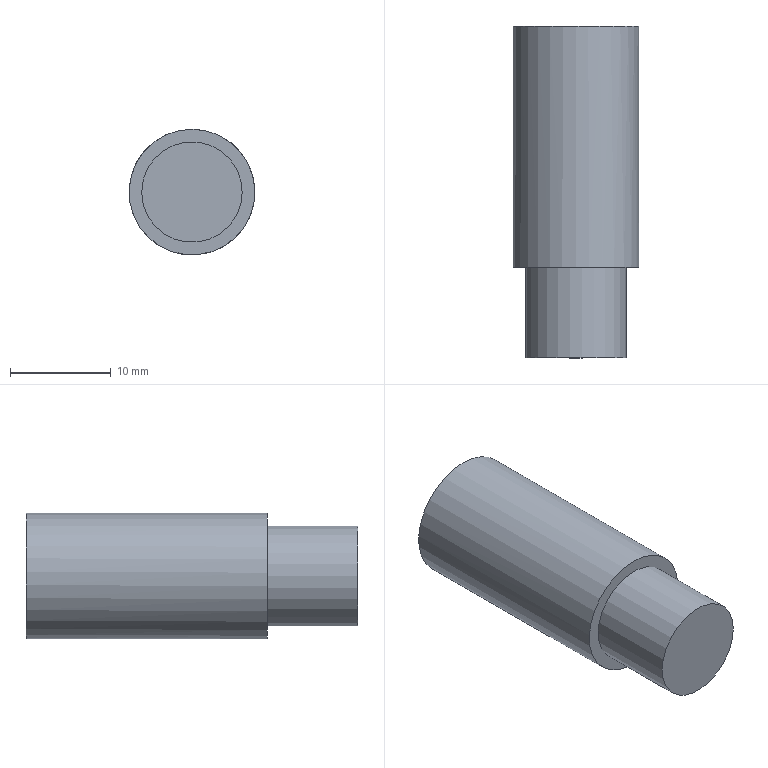Component | NX | SHORT_SHAFT | 1 solid | 5 faces | box 12.5 x 33 x 12.5 mm | volume 3652 mm3 | plane 3 | cylinder 2 | commonest cylinder face diameters 12.5 x1 10 x1
STEP:
#1=CARTESIAN_POINT('',(0.,0.,0.));
#2=DIRECTION('',(0.,0.,1.));
#3=DIRECTION('',(1.,0.,0.));
#4=AXIS2_PLACEMENT_3D('',#1,#2,#3);
#5=CARTESIAN_POINT('',(-126.826,-59.005,96.25));
#6=VERTEX_POINT('',#5);
#7=CARTESIAN_POINT('',(-126.826,-59.005,90.));
#8=DIRECTION('',(0.,1.,0.));
#9=DIRECTION('',(0.,0.,1.));
#10=AXIS2_PLACEMENT_3D('',#7,#8,#9);
#11=CIRCLE('',#10,6.25);
#12=CARTESIAN_POINT('',(-126.826,-68.005,90.));
#13=DIRECTION('',(0.,1.,0.));
#14=DIRECTION('',(0.,0.,1.));
#15=AXIS2_PLACEMENT_3D('',#12,#13,#14);
#16=CYLINDRICAL_SURFACE('',#15,6.25);
#17=CARTESIAN_POINT('',(0.,9.));
#18=DIRECTION('',(1.,0.));
#19=VECTOR('',#18,1.);
#20=LINE('',#17,#19);
#21=(GEOMETRIC_REPRESENTATION_CONTEXT(2)PARAMETRIC_REPRESENTATION_CONTEXT()REPRESENTATION_CONTEXT('',''));
#22=DEFINITIONAL_REPRESENTATION('',(#20),#21);
#23=PCURVE('',#16,#22);
#24=CARTESIAN_POINT('',(-126.826,-59.005,90.));
#25=DIRECTION('',(0.,1.,0.));
#26=DIRECTION('',(0.,0.,1.));
#27=AXIS2_PLACEMENT_3D('',#24,#25,#26);
#28=PLANE('',#27);
#29=CARTESIAN_POINT('',(0.,0.));
#30=DIRECTION('',(1.,0.));
#31=AXIS2_PLACEMENT_2D('',#29,#30);
#32=CIRCLE('',#31,6.25);
#33=(GEOMETRIC_REPRESENTATION_CONTEXT(2)PARAMETRIC_REPRESENTATION_CONTEXT()REPRESENTATION_CONTEXT('',''));
#34=DEFINITIONAL_REPRESENTATION('',(#32),#33);
#35=PCURVE('',#28,#34);
#36=SURFACE_CURVE('',#11,(#23,#35),.PCURVE_S1.);
#37=EDGE_CURVE('',#6,#6,#36,.T.);
#38=ORIENTED_EDGE('',*,*,#37,.T.);
#39=CARTESIAN_POINT('',(-126.826,-35.005,96.25));
#40=VERTEX_POINT('',#39);
#41=CARTESIAN_POINT('',(-126.826,-59.005,96.25));
#42=CARTESIAN_POINT('',(-126.826,-35.005,96.25));
#43=B_SPLINE_CURVE_WITH_KNOTS('',1,(#41,#42),.UNSPECIFIED.,.F.,.F.,(2,2),(9.,33.),.PIECEWISE_BEZIER_KNOTS.);
#44=CARTESIAN_POINT('',(6.283,0.));
#45=DIRECTION('',(0.,1.));
#46=VECTOR('',#45,1.);
#47=LINE('',#44,#46);
#48=(GEOMETRIC_REPRESENTATION_CONTEXT(2)PARAMETRIC_REPRESENTATION_CONTEXT()REPRESENTATION_CONTEXT('',''));
#49=DEFINITIONAL_REPRESENTATION('',(#47),#48);
#50=PCURVE('',#16,#49);
#51=CARTESIAN_POINT('',(0.,0.));
#52=DIRECTION('',(0.,1.));
#53=VECTOR('',#52,1.);
#54=LINE('',#51,#53);
#55=(GEOMETRIC_REPRESENTATION_CONTEXT(2)PARAMETRIC_REPRESENTATION_CONTEXT()REPRESENTATION_CONTEXT('',''));
#56=DEFINITIONAL_REPRESENTATION('',(#54),#55);
#57=PCURVE('',#16,#56);
#58=SEAM_CURVE('',#43,(#50,#57),.PCURVE_S1.);
#59=EDGE_CURVE('',#6,#40,#58,.T.);
#60=ORIENTED_EDGE('',*,*,#59,.T.);
#61=CARTESIAN_POINT('',(-120.576,-35.005,90.));
#62=VERTEX_POINT('',#61);
#63=CARTESIAN_POINT('',(-126.826,-35.005,90.));
#64=DIRECTION('',(0.,-1.,0.));
#65=DIRECTION('',(1.,0.,0.));
#66=AXIS2_PLACEMENT_3D('',#63,#64,#65);
#67=CIRCLE('',#66,6.25);
#68=CARTESIAN_POINT('',(7.854,33.));
#69=DIRECTION('',(-1.,0.));
#70=VECTOR('',#69,1.);
#71=LINE('',#68,#70);
#72=(GEOMETRIC_REPRESENTATION_CONTEXT(2)PARAMETRIC_REPRESENTATION_CONTEXT()REPRESENTATION_CONTEXT('',''));
#73=DEFINITIONAL_REPRESENTATION('',(#71),#72);
#74=PCURVE('',#16,#73);
#75=CARTESIAN_POINT('',(-126.826,-35.005,90.));
#76=DIRECTION('',(0.,-1.,0.));
#77=DIRECTION('',(0.,0.,-1.));
#78=AXIS2_PLACEMENT_3D('',#75,#76,#77);
#79=PLANE('',#78);
#80=CARTESIAN_POINT('',(0.,0.));
#81=DIRECTION('',(0.,1.));
#82=AXIS2_PLACEMENT_2D('',#80,#81);
#83=CIRCLE('',#82,6.25);
#84=(GEOMETRIC_REPRESENTATION_CONTEXT(2)PARAMETRIC_REPRESENTATION_CONTEXT()REPRESENTATION_CONTEXT('',''));
#85=DEFINITIONAL_REPRESENTATION('',(#83),#84);
#86=PCURVE('',#79,#85);
#87=SURFACE_CURVE('',#67,(#74,#86),.PCURVE_S1.);
#88=EDGE_CURVE('',#40,#62,#87,.T.);
#89=ORIENTED_EDGE('',*,*,#88,.T.);
#90=CARTESIAN_POINT('',(-126.826,-35.005,90.));
#91=DIRECTION('',(0.,-1.,0.));
#92=DIRECTION('',(1.,0.,0.));
#93=AXIS2_PLACEMENT_3D('',#90,#91,#92);
#94=CIRCLE('',#93,6.25);
#95=CARTESIAN_POINT('',(1.571,33.));
#96=DIRECTION('',(-1.,0.));
#97=VECTOR('',#96,1.);
#98=LINE('',#95,#97);
#99=(GEOMETRIC_REPRESENTATION_CONTEXT(2)PARAMETRIC_REPRESENTATION_CONTEXT()REPRESENTATION_CONTEXT('',''));
#100=DEFINITIONAL_REPRESENTATION('',(#98),#99);
#101=PCURVE('',#16,#100);
#102=CARTESIAN_POINT('',(0.,0.));
#103=DIRECTION('',(0.,1.));
#104=AXIS2_PLACEMENT_2D('',#102,#103);
#105=CIRCLE('',#104,6.25);
#106=(GEOMETRIC_REPRESENTATION_CONTEXT(2)PARAMETRIC_REPRESENTATION_CONTEXT()REPRESENTATION_CONTEXT('',''));
#107=DEFINITIONAL_REPRESENTATION('',(#105),#106);
#108=PCURVE('',#79,#107);
#109=SURFACE_CURVE('',#94,(#101,#108),.PCURVE_S1.);
#110=EDGE_CURVE('',#62,#40,#109,.T.);
#111=ORIENTED_EDGE('',*,*,#110,.T.);
#112=ORIENTED_EDGE('',*,*,#59,.F.);
#113=EDGE_LOOP('',(#38,#60,#89,#111,#112));
#114=FACE_BOUND('',#113,.T.);
#115=ADVANCED_FACE('',(#114),#16,.T.);
#116=ORIENTED_EDGE('',*,*,#110,.F.);
#117=ORIENTED_EDGE('',*,*,#88,.F.);
#118=EDGE_LOOP('',(#116,#117));
#119=FACE_BOUND('',#118,.T.);
#120=ADVANCED_FACE('',(#119),#79,.F.);
#121=CARTESIAN_POINT('',(-121.826,-59.005,90.));
#122=VERTEX_POINT('',#121);
#123=CARTESIAN_POINT('',(-126.826,-59.005,90.));
#124=DIRECTION('',(0.,-1.,0.));
#125=DIRECTION('',(1.,0.,0.));
#126=AXIS2_PLACEMENT_3D('',#123,#124,#125);
#127=CIRCLE('',#126,5.);
#128=CARTESIAN_POINT('',(0.,5.));
#129=CARTESIAN_POINT('',(8.66,5.));
#130=CARTESIAN_POINT('',(4.33,-2.5));
#131=CARTESIAN_POINT('',(0.,-10.));
#132=CARTESIAN_POINT('',(-4.33,-2.5));
#133=CARTESIAN_POINT('',(-8.66,5.));
#134=CARTESIAN_POINT('',(0.,5.));
#135=(BOUNDED_CURVE()B_SPLINE_CURVE(2,(#128,#129,#130,#131,#132,#133,#134),.UNSPECIFIED.,.T.,.F.)B_SPLINE_CURVE_WITH_KNOTS((1,2,2,2,2,1),(-2.094,0.,2.094,4.189,6.283,8.378),.UNSPECIFIED.)CURVE()GEOMETRIC_REPRESENTATION_ITEM()RATIONAL_B_SPLINE_CURVE((1.,0.5,1.,0.5,1.,0.5,1.))REPRESENTATION_ITEM(''));
#136=(GEOMETRIC_REPRESENTATION_CONTEXT(2)PARAMETRIC_REPRESENTATION_CONTEXT()REPRESENTATION_CONTEXT('',''));
#137=DEFINITIONAL_REPRESENTATION('',(#135),#136);
#138=PCURVE('',#28,#137);
#139=CARTESIAN_POINT('',(-126.826,-68.005,90.));
#140=DIRECTION('',(0.,1.,0.));
#141=DIRECTION('',(1.,0.,0.));
#142=AXIS2_PLACEMENT_3D('',#139,#140,#141);
#143=CYLINDRICAL_SURFACE('',#142,5.);
#144=CARTESIAN_POINT('',(6.283,9.));
#145=DIRECTION('',(-1.,0.));
#146=VECTOR('',#145,1.);
#147=LINE('',#144,#146);
#148=(GEOMETRIC_REPRESENTATION_CONTEXT(2)PARAMETRIC_REPRESENTATION_CONTEXT()REPRESENTATION_CONTEXT('',''));
#149=DEFINITIONAL_REPRESENTATION('',(#147),#148);
#150=PCURVE('',#143,#149);
#151=SURFACE_CURVE('',#127,(#138,#150),.PCURVE_S1.);
#152=EDGE_CURVE('',#122,#122,#151,.T.);
#153=ORIENTED_EDGE('',*,*,#152,.F.);
#154=EDGE_LOOP('',(#153));
#155=FACE_BOUND('',#154,.T.);
#156=ORIENTED_EDGE('',*,*,#37,.F.);
#157=EDGE_LOOP('',(#156));
#158=FACE_BOUND('',#157,.T.);
#159=ADVANCED_FACE('',(#155,#158),#28,.F.);
#160=CARTESIAN_POINT('',(-121.826,-68.005,90.));
#161=VERTEX_POINT('',#160);
#162=CARTESIAN_POINT('',(-126.826,-68.005,90.));
#163=DIRECTION('',(0.,1.,0.));
#164=DIRECTION('',(1.,0.,0.));
#165=AXIS2_PLACEMENT_3D('',#162,#163,#164);
#166=CIRCLE('',#165,5.);
#167=CARTESIAN_POINT('',(-126.826,-68.005,90.));
#168=DIRECTION('',(0.,-1.,0.));
#169=DIRECTION('',(0.,0.,-1.));
#170=AXIS2_PLACEMENT_3D('',#167,#168,#169);
#171=PLANE('',#170);
#172=CARTESIAN_POINT('',(0.,5.));
#173=CARTESIAN_POINT('',(8.66,5.));
#174=CARTESIAN_POINT('',(4.33,-2.5));
#175=CARTESIAN_POINT('',(0.,-10.));
#176=CARTESIAN_POINT('',(-4.33,-2.5));
#177=CARTESIAN_POINT('',(-8.66,5.));
#178=CARTESIAN_POINT('',(0.,5.));
#179=(BOUNDED_CURVE()B_SPLINE_CURVE(2,(#172,#173,#174,#175,#176,#177,#178),.UNSPECIFIED.,.T.,.F.)B_SPLINE_CURVE_WITH_KNOTS((1,2,2,2,2,1),(-2.094,0.,2.094,4.189,6.283,8.378),.UNSPECIFIED.)CURVE()GEOMETRIC_REPRESENTATION_ITEM()RATIONAL_B_SPLINE_CURVE((1.,0.5,1.,0.5,1.,0.5,1.))REPRESENTATION_ITEM(''));
#180=(GEOMETRIC_REPRESENTATION_CONTEXT(2)PARAMETRIC_REPRESENTATION_CONTEXT()REPRESENTATION_CONTEXT('',''));
#181=DEFINITIONAL_REPRESENTATION('',(#179),#180);
#182=PCURVE('',#171,#181);
#183=CARTESIAN_POINT('',(0.,0.));
#184=DIRECTION('',(1.,0.));
#185=VECTOR('',#184,1.);
#186=LINE('',#183,#185);
#187=(GEOMETRIC_REPRESENTATION_CONTEXT(2)PARAMETRIC_REPRESENTATION_CONTEXT()REPRESENTATION_CONTEXT('',''));
#188=DEFINITIONAL_REPRESENTATION('',(#186),#187);
#189=PCURVE('',#143,#188);
#190=SURFACE_CURVE('',#166,(#182,#189),.PCURVE_S1.);
#191=EDGE_CURVE('',#161,#161,#190,.T.);
#192=ORIENTED_EDGE('',*,*,#191,.F.);
#193=EDGE_LOOP('',(#192));
#194=FACE_BOUND('',#193,.T.);
#195=ADVANCED_FACE('',(#194),#171,.T.);
#196=ORIENTED_EDGE('',*,*,#152,.T.);
#197=CARTESIAN_POINT('',(-121.826,-68.005,90.));
#198=CARTESIAN_POINT('',(-121.826,-59.005,90.));
#199=B_SPLINE_CURVE_WITH_KNOTS('',1,(#197,#198),.UNSPECIFIED.,.F.,.F.,(2,2),(0.,9.),.PIECEWISE_BEZIER_KNOTS.);
#200=CARTESIAN_POINT('',(0.,0.));
#201=DIRECTION('',(0.,1.));
#202=VECTOR('',#201,1.);
#203=LINE('',#200,#202);
#204=(GEOMETRIC_REPRESENTATION_CONTEXT(2)PARAMETRIC_REPRESENTATION_CONTEXT()REPRESENTATION_CONTEXT('',''));
#205=DEFINITIONAL_REPRESENTATION('',(#203),#204);
#206=PCURVE('',#143,#205);
#207=CARTESIAN_POINT('',(6.283,0.));
#208=DIRECTION('',(0.,1.));
#209=VECTOR('',#208,1.);
#210=LINE('',#207,#209);
#211=(GEOMETRIC_REPRESENTATION_CONTEXT(2)PARAMETRIC_REPRESENTATION_CONTEXT()REPRESENTATION_CONTEXT('',''));
#212=DEFINITIONAL_REPRESENTATION('',(#210),#211);
#213=PCURVE('',#143,#212);
#214=SEAM_CURVE('',#199,(#206,#213),.PCURVE_S1.);
#215=EDGE_CURVE('',#161,#122,#214,.T.);
#216=ORIENTED_EDGE('',*,*,#215,.F.);
#217=ORIENTED_EDGE('',*,*,#191,.T.);
#218=ORIENTED_EDGE('',*,*,#215,.T.);
#219=EDGE_LOOP('',(#196,#216,#217,#218));
#220=FACE_BOUND('',#219,.T.);
#221=ADVANCED_FACE('',(#220),#143,.T.);
#222=CLOSED_SHELL('',(#115,#120,#159,#195,#221));
#223=MANIFOLD_SOLID_BREP('',#222);
#224=(LENGTH_UNIT()NAMED_UNIT(*)SI_UNIT(.MILLI.,.METRE.));
#225=UNCERTAINTY_MEASURE_WITH_UNIT(LENGTH_MEASURE(0.000005),#224,'','');
#226=(NAMED_UNIT(*)PLANE_ANGLE_UNIT()SI_UNIT($,.RADIAN.));
#227=(NAMED_UNIT(*)SI_UNIT($,.STERADIAN.)SOLID_ANGLE_UNIT());
#228=(GEOMETRIC_REPRESENTATION_CONTEXT(3)GLOBAL_UNCERTAINTY_ASSIGNED_CONTEXT((#225))GLOBAL_UNIT_ASSIGNED_CONTEXT((#224,#226,#227))REPRESENTATION_CONTEXT('',''));
#229=ADVANCED_BREP_SHAPE_REPRESENTATION('',(#4,#223),#228);